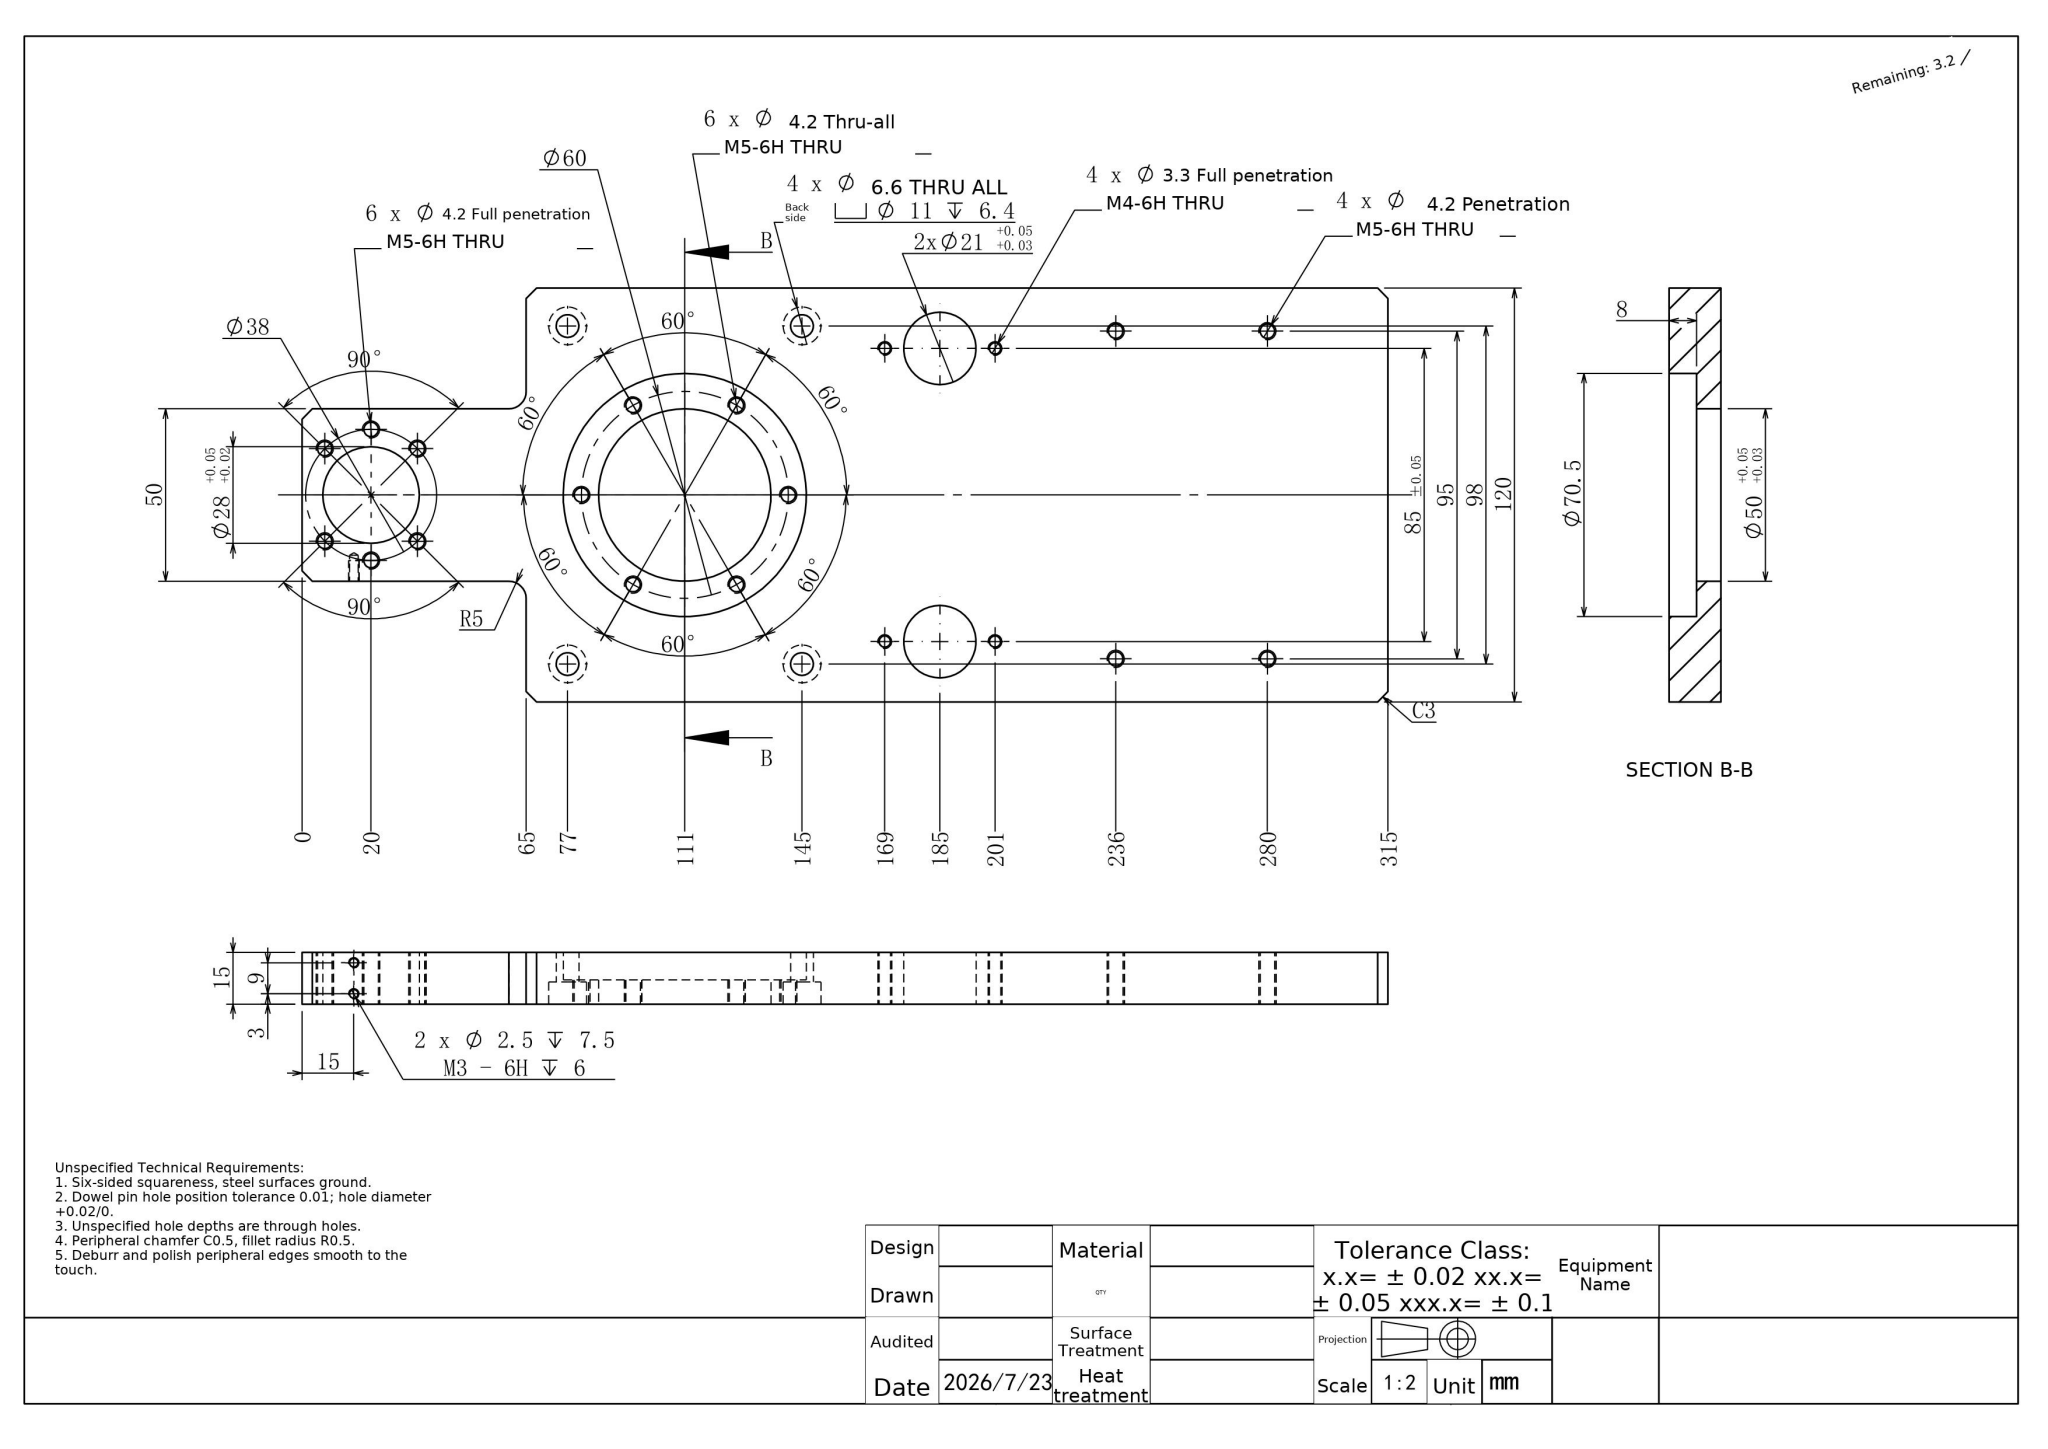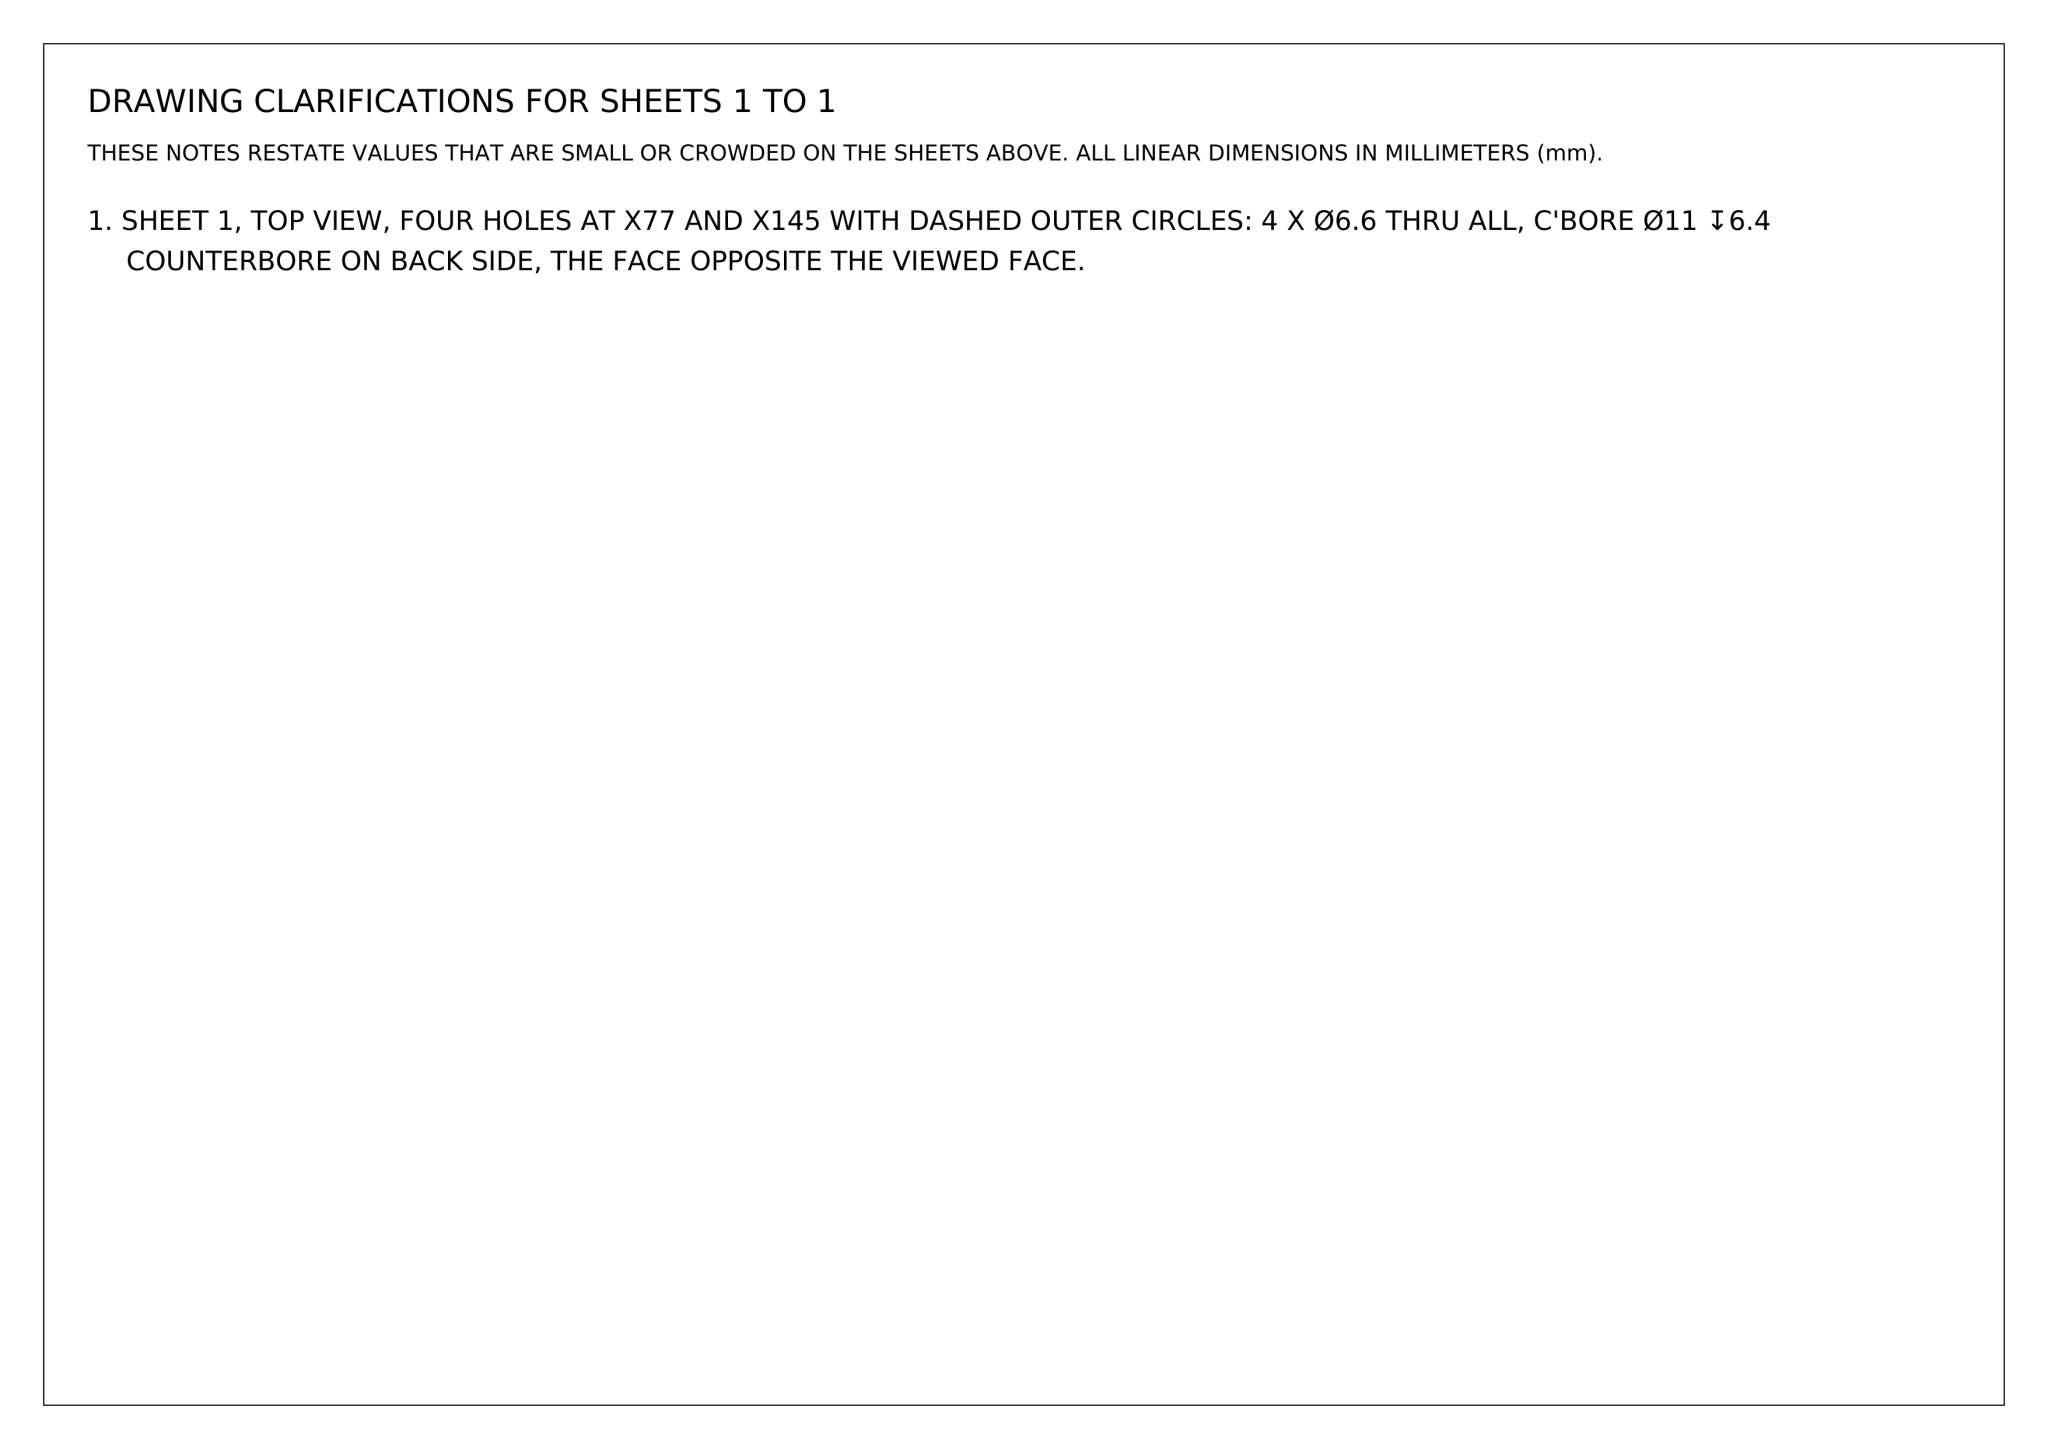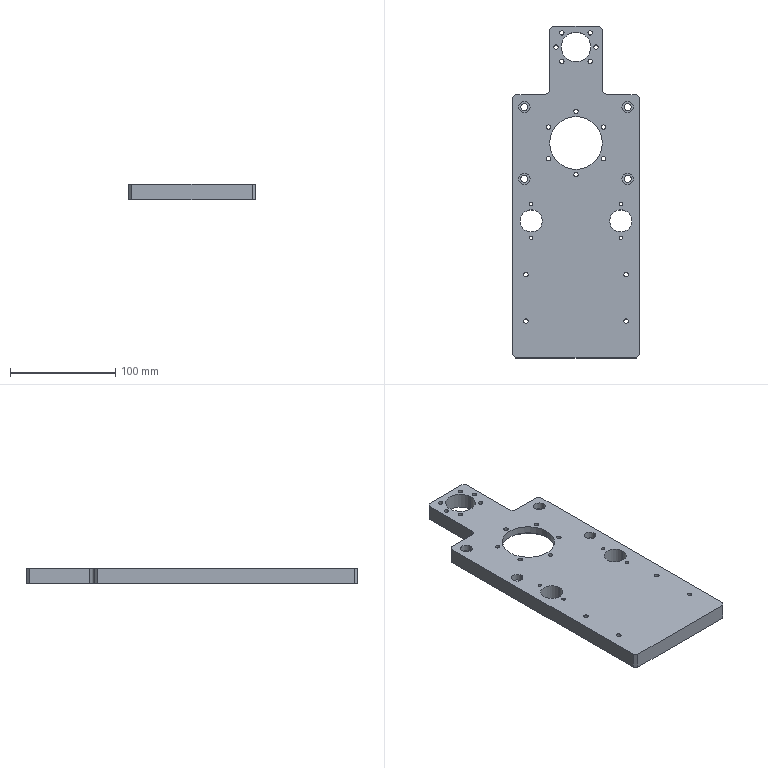Part | NX | mm | 1 solid | 97 faces | box 120 x 315 x 15 mm | volume 427046 mm3 | cylinder 72 | plane 21 | cone 4 | commonest cylinder face diameters 4.2 x32 3.3 x8 11 x8 6.6 x8 2.5 x4 21 x4 70.5 x2 28 x2